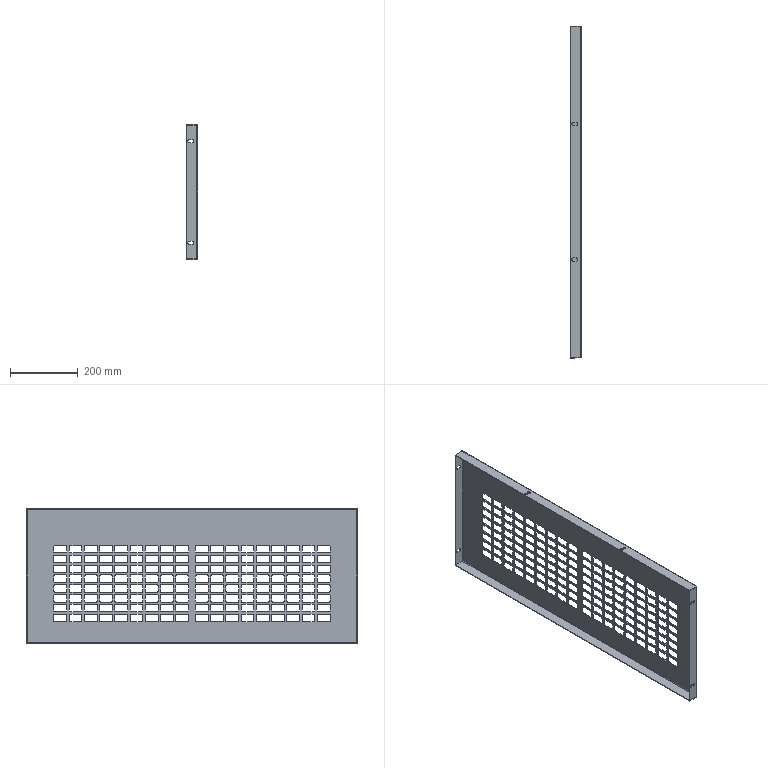Component | SolidWorks | AirInletUpperBeamAssembly-1_AirInletUpperBeam-1 | 1 solid | 1220 faces | volume 706337 mm3 | plane 610 | cylinder 602 | spline 8 | commonest cylinder face diameters 5 x576 10 x18 4 x4 8 x4 | material Plain Carbon Steel